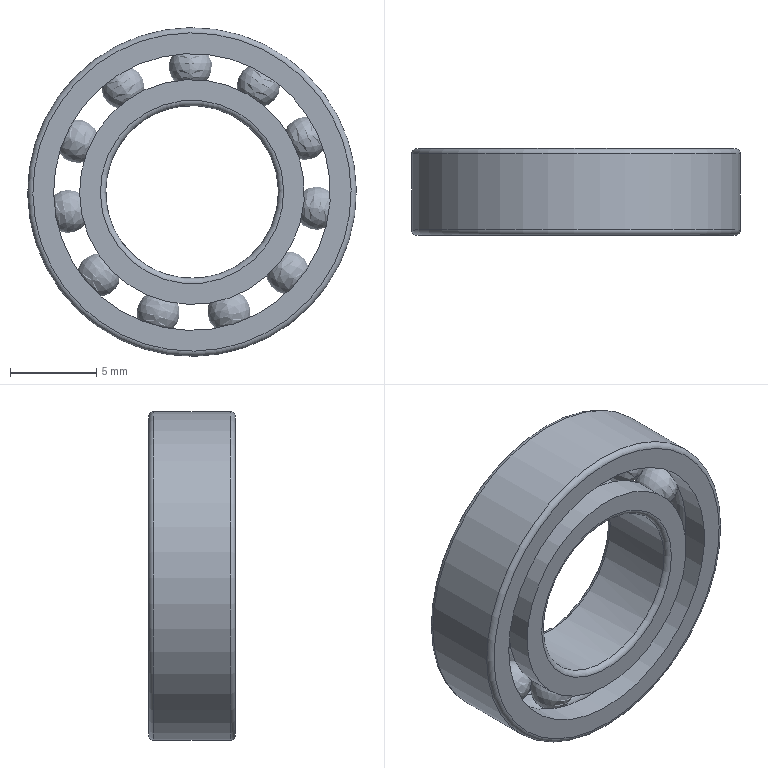Component | NX | BEARING_61800 | 13 solids | 27 faces | volume 706 mm3 | sphere 11 | cylinder 6 | torus 6 | plane 4 | commonest cylinder face diameters 16 x2 13 x2 19 x1 10 x1